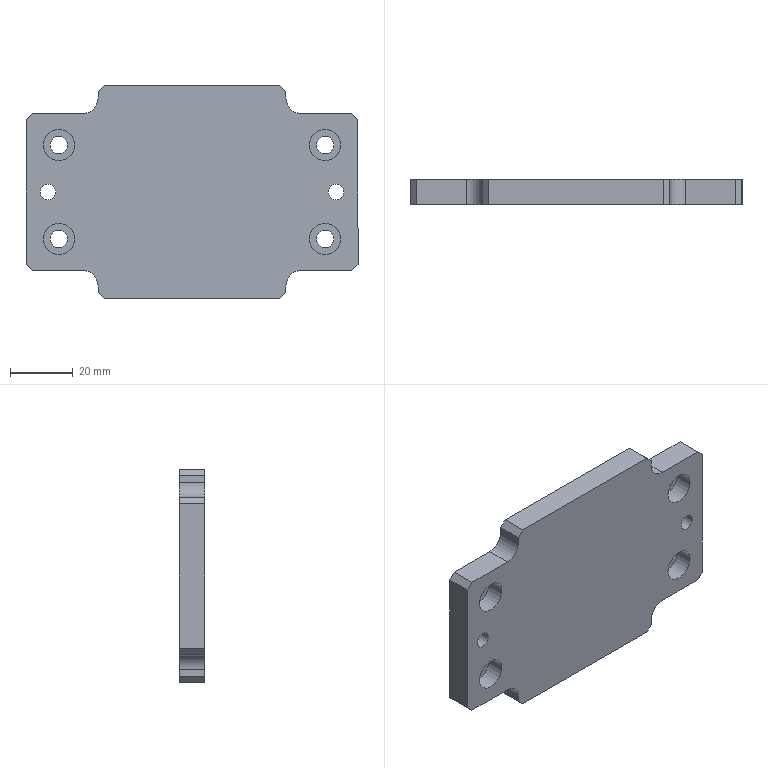Component | SolidWorks | F-SZP17248-10-04-1 | 1 solid | 50 faces | box 106 x 8 x 68 mm | volume 48760 mm3 | plane 26 | cylinder 24 | commonest cylinder face diameters 10 x12 5.5 x8 5 x4
build123d program:
from build123d import *

# Parameters (mm, degrees)
SKETCH1_W                                          = 50
SKETCH1_H                                          = 106
BOSS_EXTRUDE1_DEPTH                                = 4
HOLE_SIZE_ACCORDING_TO_TYPE_OF_HEXAGON_D           = 5.5
HOLE_SIZE_ACCORDING_TO_TYPE_OF_HEXAGON_CBORE_D     = 10
HOLE_SIZE_ACCORDING_TO_TYPE_OF_HEXAGON_CBORE_DEPTH = 5.7
SKETCH5_R                                          = 2.5
CUT_EXTRUDE1_DEPTH                                 = 60.144
SKETCH6_W                                          = 60
SKETCH6_H                                          = 8
BOSS_EXTRUDE2_DEPTH                                = 9
CHAMFER1_SIZE                                      = 2
FILLET1_R                                          = 5


with BuildPart() as part:
    # Sketch1 → Boss-Extrude1 (new, symmetric)
    with BuildSketch(Plane(origin=(0, 0, 0), x_dir=(1, 0, 0), z_dir=(0, 1, 0))):
        Rectangle(SKETCH1_W, SKETCH1_H)
    extrude(amount=BOSS_EXTRUDE1_DEPTH, both=True)

    # Hole Size_According to_ Type of Hexagon (through all)
    with Locations(Plane(origin=(0, -4, 0), x_dir=(-1, 0, 0), z_dir=(0, -1, 0))):
        with Locations((-15, -42.5), (-15, 42.5), (15, 42.5), (15, -42.5)):
            CounterBoreHole(HOLE_SIZE_ACCORDING_TO_TYPE_OF_HEXAGON_D / 2, HOLE_SIZE_ACCORDING_TO_TYPE_OF_HEXAGON_CBORE_D / 2, HOLE_SIZE_ACCORDING_TO_TYPE_OF_HEXAGON_CBORE_DEPTH)

    # Sketch5 → Cut-Extrude1 (cut, through all)
    with BuildSketch(Plane.XZ.offset(4)):
        with Locations(Location((0, 46, 0), (0, 0, 270))):
            Circle(SKETCH5_R)
        with Locations(Location((0, -46, 0), (0, 0, 270))):
            Circle(SKETCH5_R)
    extrude(amount=-CUT_EXTRUDE1_DEPTH, mode=Mode.SUBTRACT)

    # Sketch6 → Boss-Extrude2 (add)
    with BuildSketch(Plane(origin=(25, 0, 0), x_dir=(0, 0, -1), z_dir=(1, 0, 0))):
        Rectangle(SKETCH6_W, SKETCH6_H)
    boss_extrude2 = extrude(amount=BOSS_EXTRUDE2_DEPTH)

    # Mirror1: Boss-Extrude2 across plane
    add(boss_extrude2.mirror(Plane(origin=(0, 0, 0), x_dir=(0, 0, 1), z_dir=(1, 0, 0))))

    # Chamfer1
    chamfer1_edges = [part.edges().sort_by_distance(p)[0] for p in [
        (-25, 0, -53),
        (25, 0, -53),
        (25, 0, 53),
        (-25, 0, 53),
        (-34, 0, -30),
        (-34, 0, 30),
        (34, 0, -30),
        (34, 0, 30),
    ]]
    chamfer(chamfer1_edges, length=CHAMFER1_SIZE)

    # Fillet1
    fillet1_edges = [part.edges().sort_by_distance(p)[0] for p in [
        (-25, 0, 30),
        (25, 0, 30),
        (25, 0, -30),
        (-25, 0, -30),
    ]]
    fillet(fillet1_edges, radius=FILLET1_R)


solid = part.part

# Placed as in the assembly
solid = solid.moved(Location((-45.188, -34.343, 123.72), (0, 90, 0)))